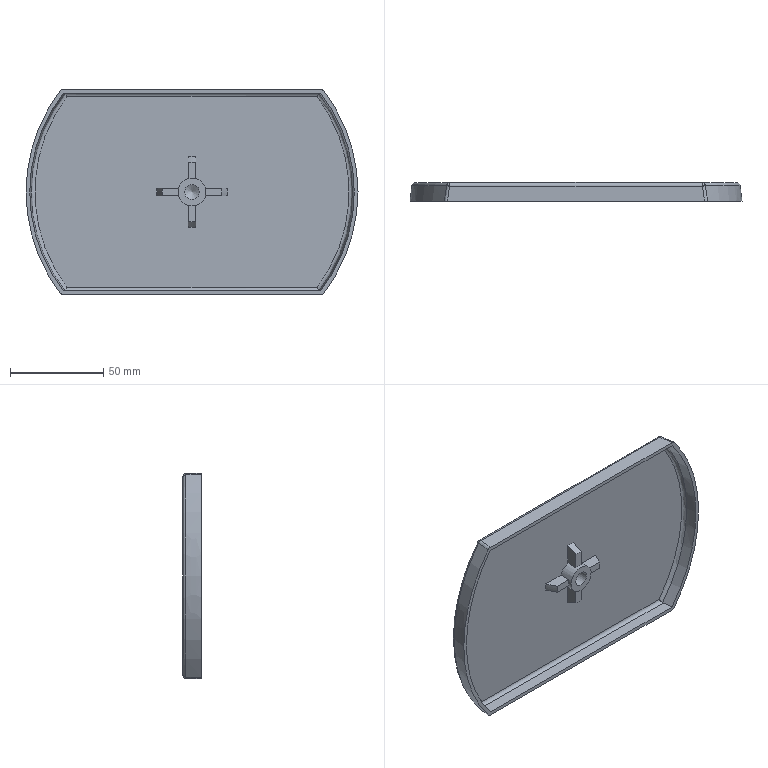Component | NX | LOWER_CASING | 1 solid | 47 faces | volume 46101 mm3 | plane 20 | spline 8 | cylinder 6 | cone 5 | torus 4 | sphere 4 | commonest cylinder face diameters 4 x4 15 x1 8 x1